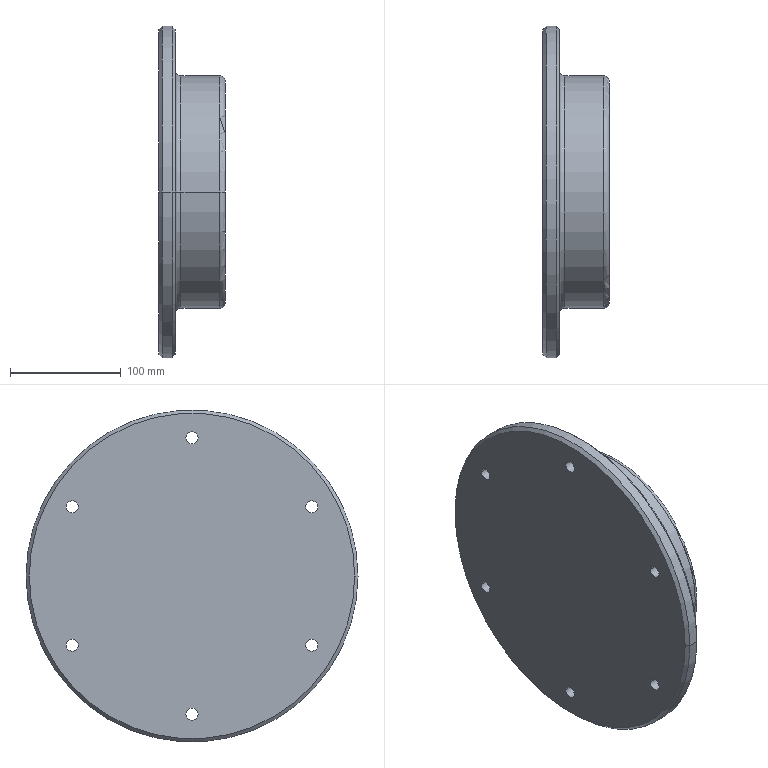Component | SolidWorks | EndCapCover-1 | 1 solid | 39 faces | box 60 x 300 x 300 mm | volume 2597910 mm3 | cone 16 | cylinder 16 | torus 4 | plane 3 | commonest cylinder face diameters 11 x12 210 x2 300 x2
STEP:
#1=COLOUR_RGB('',0.7922,0.8196,0.9333);
#2=FILL_AREA_STYLE_COLOUR('',#1);
#3=FILL_AREA_STYLE('',(#2));
#4=SURFACE_STYLE_FILL_AREA(#3);
#5=SURFACE_SIDE_STYLE('',(#4));
#6=SURFACE_STYLE_USAGE(.BOTH.,#5);
#7=PRESENTATION_STYLE_ASSIGNMENT((#6));
#8=CARTESIAN_POINT('',(4.554,30.148,43.951));
#9=VERTEX_POINT('',#8);
#10=CARTESIAN_POINT('',(4.554,38.416,43.951));
#11=VERTEX_POINT('',#10);
#12=CARTESIAN_POINT('',(4.554,34.282,43.951));
#13=DIRECTION('',(-1.,0.,0.));
#14=DIRECTION('',(0.,1.,0.));
#15=AXIS2_PLACEMENT_3D('',#12,#13,#14);
#16=CIRCLE('',#15,4.134);
#17=EDGE_CURVE('',#9,#11,#16,.T.);
#18=ORIENTED_EDGE('',*,*,#17,.F.);
#19=CARTESIAN_POINT('',(4.751,30.345,43.951));
#20=VERTEX_POINT('',#19);
#21=CARTESIAN_POINT('',(4.554,30.345,43.951));
#22=DIRECTION('',(0.,0.,1.));
#23=DIRECTION('',(0.,-1.,0.));
#24=AXIS2_PLACEMENT_3D('',#21,#22,#23);
#25=CIRCLE('',#24,0.1969);
#26=EDGE_CURVE('',#9,#20,#25,.T.);
#27=ORIENTED_EDGE('',*,*,#26,.T.);
#28=CARTESIAN_POINT('',(4.751,38.219,43.951));
#29=VERTEX_POINT('',#28);
#30=CARTESIAN_POINT('',(4.751,34.282,43.951));
#31=DIRECTION('',(1.,0.,0.));
#32=DIRECTION('',(0.,1.,0.));
#33=AXIS2_PLACEMENT_3D('',#30,#31,#32);
#34=CIRCLE('',#33,3.937);
#35=EDGE_CURVE('',#29,#20,#34,.T.);
#36=ORIENTED_EDGE('',*,*,#35,.F.);
#37=CARTESIAN_POINT('',(4.554,38.219,43.951));
#38=DIRECTION('',(0.,0.,-1.));
#39=DIRECTION('',(-1.,0.,0.));
#40=AXIS2_PLACEMENT_3D('',#37,#38,#39);
#41=CIRCLE('',#40,0.1969);
#42=EDGE_CURVE('',#11,#29,#41,.T.);
#43=ORIENTED_EDGE('',*,*,#42,.F.);
#44=EDGE_LOOP('',(#18,#27,#36,#43));
#45=FACE_OUTER_BOUND('',#44,.T.);
#46=CARTESIAN_POINT('',(4.554,34.282,43.951));
#47=DIRECTION('',(1.,0.,0.));
#48=DIRECTION('',(0.,1.,0.));
#49=AXIS2_PLACEMENT_3D('',#46,#47,#48);
#50=TOROIDAL_SURFACE('',#49,3.937,0.1969);
#51=ADVANCED_FACE('',(#45),#50,.T.);
#52=CARTESIAN_POINT('',(3.176,30.148,43.951));
#53=VERTEX_POINT('',#52);
#54=CARTESIAN_POINT('',(3.176,38.416,43.951));
#55=VERTEX_POINT('',#54);
#56=CARTESIAN_POINT('',(3.176,34.282,43.951));
#57=DIRECTION('',(1.,0.,0.));
#58=DIRECTION('',(0.,1.,0.));
#59=AXIS2_PLACEMENT_3D('',#56,#57,#58);
#60=CIRCLE('',#59,4.134);
#61=EDGE_CURVE('',#53,#55,#60,.T.);
#62=ORIENTED_EDGE('',*,*,#61,.F.);
#63=CARTESIAN_POINT('',(2.979,29.952,43.951));
#64=VERTEX_POINT('',#63);
#65=CARTESIAN_POINT('',(3.176,29.952,43.951));
#66=DIRECTION('',(0.,0.,1.));
#67=DIRECTION('',(0.,-1.,0.));
#68=AXIS2_PLACEMENT_3D('',#65,#66,#67);
#69=CIRCLE('',#68,0.1969);
#70=EDGE_CURVE('',#53,#64,#69,.T.);
#71=ORIENTED_EDGE('',*,*,#70,.T.);
#72=CARTESIAN_POINT('',(2.979,38.613,43.951));
#73=VERTEX_POINT('',#72);
#74=CARTESIAN_POINT('',(2.979,34.282,43.951));
#75=DIRECTION('',(-1.,0.,0.));
#76=DIRECTION('',(0.,1.,0.));
#77=AXIS2_PLACEMENT_3D('',#74,#75,#76);
#78=CIRCLE('',#77,4.331);
#79=EDGE_CURVE('',#73,#64,#78,.T.);
#80=ORIENTED_EDGE('',*,*,#79,.F.);
#81=CARTESIAN_POINT('',(3.176,38.613,43.951));
#82=DIRECTION('',(0.,0.,-1.));
#83=DIRECTION('',(-1.,0.,0.));
#84=AXIS2_PLACEMENT_3D('',#81,#82,#83);
#85=CIRCLE('',#84,0.1969);
#86=EDGE_CURVE('',#55,#73,#85,.T.);
#87=ORIENTED_EDGE('',*,*,#86,.F.);
#88=EDGE_LOOP('',(#62,#71,#80,#87));
#89=FACE_OUTER_BOUND('',#88,.T.);
#90=CARTESIAN_POINT('',(3.176,34.282,43.951));
#91=DIRECTION('',(1.,0.,0.));
#92=DIRECTION('',(0.,1.,0.));
#93=AXIS2_PLACEMENT_3D('',#90,#91,#92);
#94=TOROIDAL_SURFACE('',#93,4.331,0.1969);
#95=ADVANCED_FACE('',(#89),#94,.F.);
#96=CARTESIAN_POINT('',(2.979,40.07,43.951));
#97=VERTEX_POINT('',#96);
#98=CARTESIAN_POINT('',(2.979,28.495,43.951));
#99=VERTEX_POINT('',#98);
#100=CARTESIAN_POINT('',(2.979,34.282,43.951));
#101=DIRECTION('',(1.,0.,0.));
#102=DIRECTION('',(0.,1.,0.));
#103=AXIS2_PLACEMENT_3D('',#100,#101,#102);
#104=CIRCLE('',#103,5.787);
#105=EDGE_CURVE('',#97,#99,#104,.T.);
#106=ORIENTED_EDGE('',*,*,#105,.F.);
#107=CARTESIAN_POINT('',(2.861,40.188,43.951));
#108=VERTEX_POINT('',#107);
#109=CARTESIAN_POINT('',(2.861,40.188,43.951));
#110=DIRECTION('',(-0.7071,0.7071,0.));
#111=VECTOR('',#110,39.37);
#112=LINE('',#109,#111);
#113=EDGE_CURVE('',#97,#108,#112,.T.);
#114=ORIENTED_EDGE('',*,*,#113,.T.);
#115=CARTESIAN_POINT('',(2.861,28.377,43.951));
#116=VERTEX_POINT('',#115);
#117=CARTESIAN_POINT('',(2.861,34.282,43.951));
#118=DIRECTION('',(-1.,0.,0.));
#119=DIRECTION('',(0.,1.,0.));
#120=AXIS2_PLACEMENT_3D('',#117,#118,#119);
#121=CIRCLE('',#120,5.906);
#122=EDGE_CURVE('',#116,#108,#121,.T.);
#123=ORIENTED_EDGE('',*,*,#122,.F.);
#124=CARTESIAN_POINT('',(2.861,28.377,43.951));
#125=DIRECTION('',(-0.7071,-0.7071,0.));
#126=VECTOR('',#125,39.37);
#127=LINE('',#124,#126);
#128=EDGE_CURVE('',#99,#116,#127,.T.);
#129=ORIENTED_EDGE('',*,*,#128,.F.);
#130=EDGE_LOOP('',(#106,#114,#123,#129));
#131=FACE_OUTER_BOUND('',#130,.T.);
#132=CARTESIAN_POINT('',(2.861,34.282,43.951));
#133=DIRECTION('',(-1.,0.,0.));
#134=DIRECTION('',(0.,-1.,0.));
#135=AXIS2_PLACEMENT_3D('',#132,#133,#134);
#136=CONICAL_SURFACE('',#135,5.906,0.7854);
#137=ADVANCED_FACE('',(#131),#136,.T.);
#138=CARTESIAN_POINT('',(2.388,28.495,43.951));
#139=VERTEX_POINT('',#138);
#140=CARTESIAN_POINT('',(2.388,40.07,43.951));
#141=VERTEX_POINT('',#140);
#142=CARTESIAN_POINT('',(2.388,34.282,43.951));
#143=DIRECTION('',(-1.,0.,0.));
#144=DIRECTION('',(0.,-1.,0.));
#145=AXIS2_PLACEMENT_3D('',#142,#143,#144);
#146=CIRCLE('',#145,5.787);
#147=EDGE_CURVE('',#139,#141,#146,.T.);
#148=ORIENTED_EDGE('',*,*,#147,.F.);
#149=CARTESIAN_POINT('',(2.507,28.377,43.951));
#150=VERTEX_POINT('',#149);
#151=CARTESIAN_POINT('',(2.388,28.495,43.951));
#152=DIRECTION('',(0.7071,-0.7071,0.));
#153=VECTOR('',#152,39.37);
#154=LINE('',#151,#153);
#155=EDGE_CURVE('',#139,#150,#154,.T.);
#156=ORIENTED_EDGE('',*,*,#155,.T.);
#157=CARTESIAN_POINT('',(2.507,40.188,43.951));
#158=VERTEX_POINT('',#157);
#159=CARTESIAN_POINT('',(2.507,34.282,43.951));
#160=DIRECTION('',(1.,0.,0.));
#161=DIRECTION('',(0.,-1.,0.));
#162=AXIS2_PLACEMENT_3D('',#159,#160,#161);
#163=CIRCLE('',#162,5.906);
#164=EDGE_CURVE('',#158,#150,#163,.T.);
#165=ORIENTED_EDGE('',*,*,#164,.F.);
#166=CARTESIAN_POINT('',(2.388,40.07,43.951));
#167=DIRECTION('',(0.7071,0.7071,0.));
#168=VECTOR('',#167,39.37);
#169=LINE('',#166,#168);
#170=EDGE_CURVE('',#141,#158,#169,.T.);
#171=ORIENTED_EDGE('',*,*,#170,.F.);
#172=EDGE_LOOP('',(#148,#156,#165,#171));
#173=FACE_OUTER_BOUND('',#172,.T.);
#174=CARTESIAN_POINT('',(2.388,34.282,43.951));
#175=DIRECTION('',(1.,0.,0.));
#176=DIRECTION('',(0.,1.,0.));
#177=AXIS2_PLACEMENT_3D('',#174,#175,#176);
#178=CONICAL_SURFACE('',#177,5.787,0.7854);
#179=ADVANCED_FACE('',(#173),#178,.T.);
#180=CARTESIAN_POINT('',(2.764,38.322,46.408));
#181=VERTEX_POINT('',#180);
#182=CARTESIAN_POINT('',(2.764,38.755,46.408));
#183=VERTEX_POINT('',#182);
#184=CARTESIAN_POINT('',(2.764,38.538,46.408));
#185=DIRECTION('',(1.,0.,0.));
#186=DIRECTION('',(0.,1.,0.));
#187=AXIS2_PLACEMENT_3D('',#184,#185,#186);
#188=CIRCLE('',#187,0.2165);
#189=EDGE_CURVE('',#181,#183,#188,.T.);
#190=ORIENTED_EDGE('',*,*,#189,.F.);
#191=CARTESIAN_POINT('',(2.979,38.107,46.408));
#192=VERTEX_POINT('',#191);
#193=CARTESIAN_POINT('',(2.764,38.322,46.408));
#194=DIRECTION('',(0.7071,-0.7071,0.));
#195=VECTOR('',#194,39.37);
#196=LINE('',#193,#195);
#197=EDGE_CURVE('',#181,#192,#196,.T.);
#198=ORIENTED_EDGE('',*,*,#197,.T.);
#199=CARTESIAN_POINT('',(2.979,38.969,46.408));
#200=VERTEX_POINT('',#199);
#201=CARTESIAN_POINT('',(2.979,38.538,46.408));
#202=DIRECTION('',(-1.,0.,0.));
#203=DIRECTION('',(0.,1.,0.));
#204=AXIS2_PLACEMENT_3D('',#201,#202,#203);
#205=CIRCLE('',#204,0.4311);
#206=EDGE_CURVE('',#200,#192,#205,.T.);
#207=ORIENTED_EDGE('',*,*,#206,.F.);
#208=CARTESIAN_POINT('',(2.764,38.755,46.408));
#209=DIRECTION('',(0.7071,0.7071,0.));
#210=VECTOR('',#209,39.37);
#211=LINE('',#208,#210);
#212=EDGE_CURVE('',#183,#200,#211,.T.);
#213=ORIENTED_EDGE('',*,*,#212,.F.);
#214=EDGE_LOOP('',(#190,#198,#207,#213));
#215=FACE_OUTER_BOUND('',#214,.T.);
#216=CARTESIAN_POINT('',(2.764,38.538,46.408));
#217=DIRECTION('',(1.,0.,0.));
#218=DIRECTION('',(0.,1.,0.));
#219=AXIS2_PLACEMENT_3D('',#216,#217,#218);
#220=CONICAL_SURFACE('',#219,0.2165,0.7854);
#221=ADVANCED_FACE('',(#215),#220,.F.);
#222=CARTESIAN_POINT('',(2.764,34.066,48.865));
#223=VERTEX_POINT('',#222);
#224=CARTESIAN_POINT('',(2.764,34.499,48.865));
#225=VERTEX_POINT('',#224);
#226=CARTESIAN_POINT('',(2.764,34.282,48.865));
#227=DIRECTION('',(1.,0.,0.));
#228=DIRECTION('',(0.,1.,0.));
#229=AXIS2_PLACEMENT_3D('',#226,#227,#228);
#230=CIRCLE('',#229,0.2165);
#231=EDGE_CURVE('',#223,#225,#230,.T.);
#232=ORIENTED_EDGE('',*,*,#231,.F.);
#233=CARTESIAN_POINT('',(2.979,33.851,48.865));
#234=VERTEX_POINT('',#233);
#235=CARTESIAN_POINT('',(2.764,34.066,48.865));
#236=DIRECTION('',(0.7071,-0.7071,0.));
#237=VECTOR('',#236,39.37);
#238=LINE('',#235,#237);
#239=EDGE_CURVE('',#223,#234,#238,.T.);
#240=ORIENTED_EDGE('',*,*,#239,.T.);
#241=CARTESIAN_POINT('',(2.979,34.713,48.865));
#242=VERTEX_POINT('',#241);
#243=CARTESIAN_POINT('',(2.979,34.282,48.865));
#244=DIRECTION('',(-1.,0.,0.));
#245=DIRECTION('',(0.,1.,0.));
#246=AXIS2_PLACEMENT_3D('',#243,#244,#245);
#247=CIRCLE('',#246,0.4311);
#248=EDGE_CURVE('',#242,#234,#247,.T.);
#249=ORIENTED_EDGE('',*,*,#248,.F.);
#250=CARTESIAN_POINT('',(2.764,34.499,48.865));
#251=DIRECTION('',(0.7071,0.7071,0.));
#252=VECTOR('',#251,39.37);
#253=LINE('',#250,#252);
#254=EDGE_CURVE('',#225,#242,#253,.T.);
#255=ORIENTED_EDGE('',*,*,#254,.F.);
#256=EDGE_LOOP('',(#232,#240,#249,#255));
#257=FACE_OUTER_BOUND('',#256,.T.);
#258=CARTESIAN_POINT('',(2.764,34.282,48.865));
#259=DIRECTION('',(1.,0.,0.));
#260=DIRECTION('',(0.,1.,0.));
#261=AXIS2_PLACEMENT_3D('',#258,#259,#260);
#262=CONICAL_SURFACE('',#261,0.2165,0.7854);
#263=ADVANCED_FACE('',(#257),#262,.F.);
#264=CARTESIAN_POINT('',(2.764,29.81,41.494));
#265=VERTEX_POINT('',#264);
#266=CARTESIAN_POINT('',(2.764,30.243,41.494));
#267=VERTEX_POINT('',#266);
#268=CARTESIAN_POINT('',(2.764,30.026,41.494));
#269=DIRECTION('',(1.,0.,0.));
#270=DIRECTION('',(0.,1.,0.));
#271=AXIS2_PLACEMENT_3D('',#268,#269,#270);
#272=CIRCLE('',#271,0.2165);
#273=EDGE_CURVE('',#265,#267,#272,.T.);
#274=ORIENTED_EDGE('',*,*,#273,.F.);
#275=CARTESIAN_POINT('',(2.979,29.595,41.494));
#276=VERTEX_POINT('',#275);
#277=CARTESIAN_POINT('',(2.764,29.81,41.494));
#278=DIRECTION('',(0.7071,-0.7071,0.));
#279=VECTOR('',#278,39.37);
#280=LINE('',#277,#279);
#281=EDGE_CURVE('',#265,#276,#280,.T.);
#282=ORIENTED_EDGE('',*,*,#281,.T.);
#283=CARTESIAN_POINT('',(2.979,30.457,41.494));
#284=VERTEX_POINT('',#283);
#285=CARTESIAN_POINT('',(2.979,30.026,41.494));
#286=DIRECTION('',(-1.,0.,0.));
#287=DIRECTION('',(0.,1.,0.));
#288=AXIS2_PLACEMENT_3D('',#285,#286,#287);
#289=CIRCLE('',#288,0.4311);
#290=EDGE_CURVE('',#284,#276,#289,.T.);
#291=ORIENTED_EDGE('',*,*,#290,.F.);
#292=CARTESIAN_POINT('',(2.764,30.243,41.494));
#293=DIRECTION('',(0.7071,0.7071,0.));
#294=VECTOR('',#293,39.37);
#295=LINE('',#292,#294);
#296=EDGE_CURVE('',#267,#284,#295,.T.);
#297=ORIENTED_EDGE('',*,*,#296,.F.);
#298=EDGE_LOOP('',(#274,#282,#291,#297));
#299=FACE_OUTER_BOUND('',#298,.T.);
#300=CARTESIAN_POINT('',(2.764,30.026,41.494));
#301=DIRECTION('',(1.,0.,0.));
#302=DIRECTION('',(0.,1.,0.));
#303=AXIS2_PLACEMENT_3D('',#300,#301,#302);
#304=CONICAL_SURFACE('',#303,0.2165,0.7854);
#305=ADVANCED_FACE('',(#299),#304,.F.);
#306=CARTESIAN_POINT('',(2.764,34.066,39.036));
#307=VERTEX_POINT('',#306);
#308=CARTESIAN_POINT('',(2.764,34.499,39.036));
#309=VERTEX_POINT('',#308);
#310=CARTESIAN_POINT('',(2.764,34.282,39.036));
#311=DIRECTION('',(1.,0.,0.));
#312=DIRECTION('',(0.,1.,0.));
#313=AXIS2_PLACEMENT_3D('',#310,#311,#312);
#314=CIRCLE('',#313,0.2165);
#315=EDGE_CURVE('',#307,#309,#314,.T.);
#316=ORIENTED_EDGE('',*,*,#315,.F.);
#317=CARTESIAN_POINT('',(2.979,33.851,39.036));
#318=VERTEX_POINT('',#317);
#319=CARTESIAN_POINT('',(2.764,34.066,39.036));
#320=DIRECTION('',(0.7071,-0.7071,0.));
#321=VECTOR('',#320,39.37);
#322=LINE('',#319,#321);
#323=EDGE_CURVE('',#307,#318,#322,.T.);
#324=ORIENTED_EDGE('',*,*,#323,.T.);
#325=CARTESIAN_POINT('',(2.979,34.713,39.036));
#326=VERTEX_POINT('',#325);
#327=CARTESIAN_POINT('',(2.979,34.282,39.036));
#328=DIRECTION('',(-1.,0.,0.));
#329=DIRECTION('',(0.,1.,0.));
#330=AXIS2_PLACEMENT_3D('',#327,#328,#329);
#331=CIRCLE('',#330,0.4311);
#332=EDGE_CURVE('',#326,#318,#331,.T.);
#333=ORIENTED_EDGE('',*,*,#332,.F.);
#334=CARTESIAN_POINT('',(2.764,34.499,39.036));
#335=DIRECTION('',(0.7071,0.7071,0.));
#336=VECTOR('',#335,39.37);
#337=LINE('',#334,#336);
#338=EDGE_CURVE('',#309,#326,#337,.T.);
#339=ORIENTED_EDGE('',*,*,#338,.F.);
#340=EDGE_LOOP('',(#316,#324,#333,#339));
#341=FACE_OUTER_BOUND('',#340,.T.);
#342=CARTESIAN_POINT('',(2.764,34.282,39.036));
#343=DIRECTION('',(1.,0.,0.));
#344=DIRECTION('',(0.,1.,0.));
#345=AXIS2_PLACEMENT_3D('',#342,#343,#344);
#346=CONICAL_SURFACE('',#345,0.2165,0.7854);
#347=ADVANCED_FACE('',(#341),#346,.F.);
#348=CARTESIAN_POINT('',(2.764,29.81,46.408));
#349=VERTEX_POINT('',#348);
#350=CARTESIAN_POINT('',(2.764,30.243,46.408));
#351=VERTEX_POINT('',#350);
#352=CARTESIAN_POINT('',(2.764,30.026,46.408));
#353=DIRECTION('',(1.,0.,0.));
#354=DIRECTION('',(0.,1.,0.));
#355=AXIS2_PLACEMENT_3D('',#352,#353,#354);
#356=CIRCLE('',#355,0.2165);
#357=EDGE_CURVE('',#349,#351,#356,.T.);
#358=ORIENTED_EDGE('',*,*,#357,.F.);
#359=CARTESIAN_POINT('',(2.979,29.595,46.408));
#360=VERTEX_POINT('',#359);
#361=CARTESIAN_POINT('',(2.764,29.81,46.408));
#362=DIRECTION('',(0.7071,-0.7071,0.));
#363=VECTOR('',#362,39.37);
#364=LINE('',#361,#363);
#365=EDGE_CURVE('',#349,#360,#364,.T.);
#366=ORIENTED_EDGE('',*,*,#365,.T.);
#367=CARTESIAN_POINT('',(2.979,30.457,46.408));
#368=VERTEX_POINT('',#367);
#369=CARTESIAN_POINT('',(2.979,30.026,46.408));
#370=DIRECTION('',(-1.,0.,0.));
#371=DIRECTION('',(0.,1.,0.));
#372=AXIS2_PLACEMENT_3D('',#369,#370,#371);
#373=CIRCLE('',#372,0.4311);
#374=EDGE_CURVE('',#368,#360,#373,.T.);
#375=ORIENTED_EDGE('',*,*,#374,.F.);
#376=CARTESIAN_POINT('',(2.764,30.243,46.408));
#377=DIRECTION('',(0.7071,0.7071,0.));
#378=VECTOR('',#377,39.37);
#379=LINE('',#376,#378);
#380=EDGE_CURVE('',#351,#368,#379,.T.);
#381=ORIENTED_EDGE('',*,*,#380,.F.);
#382=EDGE_LOOP('',(#358,#366,#375,#381));
#383=FACE_OUTER_BOUND('',#382,.T.);
#384=CARTESIAN_POINT('',(2.764,30.026,46.408));
#385=DIRECTION('',(1.,0.,0.));
#386=DIRECTION('',(0.,1.,0.));
#387=AXIS2_PLACEMENT_3D('',#384,#385,#386);
#388=CONICAL_SURFACE('',#387,0.2165,0.7854);
#389=ADVANCED_FACE('',(#383),#388,.F.);
#390=CARTESIAN_POINT('',(2.764,38.322,41.494));
#391=VERTEX_POINT('',#390);
#392=CARTESIAN_POINT('',(2.764,38.755,41.494));
#393=VERTEX_POINT('',#392);
#394=CARTESIAN_POINT('',(2.764,38.538,41.494));
#395=DIRECTION('',(1.,0.,0.));
#396=DIRECTION('',(0.,1.,0.));
#397=AXIS2_PLACEMENT_3D('',#394,#395,#396);
#398=CIRCLE('',#397,0.2165);
#399=EDGE_CURVE('',#391,#393,#398,.T.);
#400=ORIENTED_EDGE('',*,*,#399,.F.);
#401=CARTESIAN_POINT('',(2.979,38.107,41.494));
#402=VERTEX_POINT('',#401);
#403=CARTESIAN_POINT('',(2.764,38.322,41.494));
#404=DIRECTION('',(0.7071,-0.7071,0.));
#405=VECTOR('',#404,39.37);
#406=LINE('',#403,#405);
#407=EDGE_CURVE('',#391,#402,#406,.T.);
#408=ORIENTED_EDGE('',*,*,#407,.T.);
#409=CARTESIAN_POINT('',(2.979,38.969,41.494));
#410=VERTEX_POINT('',#409);
#411=CARTESIAN_POINT('',(2.979,38.538,41.494));
#412=DIRECTION('',(-1.,0.,0.));
#413=DIRECTION('',(0.,1.,0.));
#414=AXIS2_PLACEMENT_3D('',#411,#412,#413);
#415=CIRCLE('',#414,0.4311);
#416=EDGE_CURVE('',#410,#402,#415,.T.);
#417=ORIENTED_EDGE('',*,*,#416,.F.);
#418=CARTESIAN_POINT('',(2.764,38.755,41.494));
#419=DIRECTION('',(0.7071,0.7071,0.));
#420=VECTOR('',#419,39.37);
#421=LINE('',#418,#420);
#422=EDGE_CURVE('',#393,#410,#421,.T.);
#423=ORIENTED_EDGE('',*,*,#422,.F.);
#424=EDGE_LOOP('',(#400,#408,#417,#423));
#425=FACE_OUTER_BOUND('',#424,.T.);
#426=CARTESIAN_POINT('',(2.764,38.538,41.494));
#427=DIRECTION('',(1.,0.,0.));
#428=DIRECTION('',(0.,1.,0.));
#429=AXIS2_PLACEMENT_3D('',#426,#427,#428);
#430=CONICAL_SURFACE('',#429,0.2165,0.7854);
#431=ADVANCED_FACE('',(#425),#430,.F.);
#432=CARTESIAN_POINT('',(2.388,29.81,41.494));
#433=VERTEX_POINT('',#432);
#434=CARTESIAN_POINT('',(2.388,30.243,41.494));
#435=VERTEX_POINT('',#434);
#436=CARTESIAN_POINT('',(2.388,30.026,41.494));
#437=DIRECTION('',(1.,0.,0.));
#438=DIRECTION('',(0.,1.,0.));
#439=AXIS2_PLACEMENT_3D('',#436,#437,#438);
#440=CIRCLE('',#439,0.2165);
#441=EDGE_CURVE('',#433,#435,#440,.T.);
#442=ORIENTED_EDGE('',*,*,#441,.F.);
#443=CARTESIAN_POINT('',(2.979,29.81,41.494));
#444=DIRECTION('',(1.,0.,0.));
#445=VECTOR('',#444,39.37);
#446=LINE('',#443,#445);
#447=EDGE_CURVE('',#433,#265,#446,.T.);
#448=ORIENTED_EDGE('',*,*,#447,.T.);
#449=ORIENTED_EDGE('',*,*,#273,.T.);
#450=CARTESIAN_POINT('',(2.979,30.243,41.494));
#451=DIRECTION('',(1.,0.,0.));
#452=VECTOR('',#451,39.37);
#453=LINE('',#450,#452);
#454=EDGE_CURVE('',#435,#267,#453,.T.);
#455=ORIENTED_EDGE('',*,*,#454,.F.);
#456=EDGE_LOOP('',(#442,#448,#449,#455));
#457=FACE_OUTER_BOUND('',#456,.T.);
#458=CARTESIAN_POINT('',(2.979,30.026,41.494));
#459=DIRECTION('',(1.,0.,0.));
#460=DIRECTION('',(0.,1.,0.));
#461=AXIS2_PLACEMENT_3D('',#458,#459,#460);
#462=CYLINDRICAL_SURFACE('',#461,0.2165);
#463=ADVANCED_FACE('',(#457),#462,.F.);
#464=CARTESIAN_POINT('',(2.388,29.81,46.408));
#465=VERTEX_POINT('',#464);
#466=CARTESIAN_POINT('',(2.388,30.243,46.408));
#467=VERTEX_POINT('',#466);
#468=CARTESIAN_POINT('',(2.388,30.026,46.408));
#469=DIRECTION('',(1.,0.,0.));
#470=DIRECTION('',(0.,1.,0.));
#471=AXIS2_PLACEMENT_3D('',#468,#469,#470);
#472=CIRCLE('',#471,0.2165);
#473=EDGE_CURVE('',#465,#467,#472,.T.);
#474=ORIENTED_EDGE('',*,*,#473,.F.);
#475=CARTESIAN_POINT('',(2.979,29.81,46.408));
#476=DIRECTION('',(1.,0.,0.));
#477=VECTOR('',#476,39.37);
#478=LINE('',#475,#477);
#479=EDGE_CURVE('',#465,#349,#478,.T.);
#480=ORIENTED_EDGE('',*,*,#479,.T.);
#481=ORIENTED_EDGE('',*,*,#357,.T.);
#482=CARTESIAN_POINT('',(2.979,30.243,46.408));
#483=DIRECTION('',(1.,0.,0.));
#484=VECTOR('',#483,39.37);
#485=LINE('',#482,#484);
#486=EDGE_CURVE('',#467,#351,#485,.T.);
#487=ORIENTED_EDGE('',*,*,#486,.F.);
#488=EDGE_LOOP('',(#474,#480,#481,#487));
#489=FACE_OUTER_BOUND('',#488,.T.);
#490=CARTESIAN_POINT('',(2.979,30.026,46.408));
#491=DIRECTION('',(1.,0.,0.));
#492=DIRECTION('',(0.,1.,0.));
#493=AXIS2_PLACEMENT_3D('',#490,#491,#492);
#494=CYLINDRICAL_SURFACE('',#493,0.2165);
#495=ADVANCED_FACE('',(#489),#494,.F.);
#496=CARTESIAN_POINT('',(2.388,34.066,48.865));
#497=VERTEX_POINT('',#496);
#498=CARTESIAN_POINT('',(2.388,34.499,48.865));
#499=VERTEX_POINT('',#498);
#500=CARTESIAN_POINT('',(2.388,34.282,48.865));
#501=DIRECTION('',(1.,0.,0.));
#502=DIRECTION('',(0.,1.,0.));
#503=AXIS2_PLACEMENT_3D('',#500,#501,#502);
#504=CIRCLE('',#503,0.2165);
#505=EDGE_CURVE('',#497,#499,#504,.T.);
#506=ORIENTED_EDGE('',*,*,#505,.F.);
#507=CARTESIAN_POINT('',(2.979,34.066,48.865));
#508=DIRECTION('',(1.,0.,0.));
#509=VECTOR('',#508,39.37);
#510=LINE('',#507,#509);
#511=EDGE_CURVE('',#497,#223,#510,.T.);
#512=ORIENTED_EDGE('',*,*,#511,.T.);
#513=ORIENTED_EDGE('',*,*,#231,.T.);
#514=CARTESIAN_POINT('',(2.979,34.499,48.865));
#515=DIRECTION('',(1.,0.,0.));
#516=VECTOR('',#515,39.37);
#517=LINE('',#514,#516);
#518=EDGE_CURVE('',#499,#225,#517,.T.);
#519=ORIENTED_EDGE('',*,*,#518,.F.);
#520=EDGE_LOOP('',(#506,#512,#513,#519));
#521=FACE_OUTER_BOUND('',#520,.T.);
#522=CARTESIAN_POINT('',(2.979,34.282,48.865));
#523=DIRECTION('',(1.,0.,0.));
#524=DIRECTION('',(0.,1.,0.));
#525=AXIS2_PLACEMENT_3D('',#522,#523,#524);
#526=CYLINDRICAL_SURFACE('',#525,0.2165);
#527=ADVANCED_FACE('',(#521),#526,.F.);
#528=CARTESIAN_POINT('',(2.388,38.322,46.408));
#529=VERTEX_POINT('',#528);
#530=CARTESIAN_POINT('',(2.388,38.755,46.408));
#531=VERTEX_POINT('',#530);
#532=CARTESIAN_POINT('',(2.388,38.538,46.408));
#533=DIRECTION('',(1.,0.,0.));
#534=DIRECTION('',(0.,1.,0.));
#535=AXIS2_PLACEMENT_3D('',#532,#533,#534);
#536=CIRCLE('',#535,0.2165);
#537=EDGE_CURVE('',#529,#531,#536,.T.);
#538=ORIENTED_EDGE('',*,*,#537,.F.);
#539=CARTESIAN_POINT('',(2.979,38.322,46.408));
#540=DIRECTION('',(1.,0.,0.));
#541=VECTOR('',#540,39.37);
#542=LINE('',#539,#541);
#543=EDGE_CURVE('',#529,#181,#542,.T.);
#544=ORIENTED_EDGE('',*,*,#543,.T.);
#545=ORIENTED_EDGE('',*,*,#189,.T.);
#546=CARTESIAN_POINT('',(2.979,38.755,46.408));
#547=DIRECTION('',(1.,0.,0.));
#548=VECTOR('',#547,39.37);
#549=LINE('',#546,#548);
#550=EDGE_CURVE('',#531,#183,#549,.T.);
#551=ORIENTED_EDGE('',*,*,#550,.F.);
#552=EDGE_LOOP('',(#538,#544,#545,#551));
#553=FACE_OUTER_BOUND('',#552,.T.);
#554=CARTESIAN_POINT('',(2.979,38.538,46.408));
#555=DIRECTION('',(1.,0.,0.));
#556=DIRECTION('',(0.,1.,0.));
#557=AXIS2_PLACEMENT_3D('',#554,#555,#556);
#558=CYLINDRICAL_SURFACE('',#557,0.2165);
#559=ADVANCED_FACE('',(#553),#558,.F.);
#560=CARTESIAN_POINT('',(2.388,38.322,41.494));
#561=VERTEX_POINT('',#560);
#562=CARTESIAN_POINT('',(2.388,38.755,41.494));
#563=VERTEX_POINT('',#562);
#564=CARTESIAN_POINT('',(2.388,38.538,41.494));
#565=DIRECTION('',(1.,0.,0.));
#566=DIRECTION('',(0.,1.,0.));
#567=AXIS2_PLACEMENT_3D('',#564,#565,#566);
#568=CIRCLE('',#567,0.2165);
#569=EDGE_CURVE('',#561,#563,#568,.T.);
#570=ORIENTED_EDGE('',*,*,#569,.F.);
#571=CARTESIAN_POINT('',(2.979,38.322,41.494));
#572=DIRECTION('',(1.,0.,0.));
#573=VECTOR('',#572,39.37);
#574=LINE('',#571,#573);
#575=EDGE_CURVE('',#561,#391,#574,.T.);
#576=ORIENTED_EDGE('',*,*,#575,.T.);
#577=ORIENTED_EDGE('',*,*,#399,.T.);
#578=CARTESIAN_POINT('',(2.979,38.755,41.494));
#579=DIRECTION('',(1.,0.,0.));
#580=VECTOR('',#579,39.37);
#581=LINE('',#578,#580);
#582=EDGE_CURVE('',#563,#393,#581,.T.);
#583=ORIENTED_EDGE('',*,*,#582,.F.);
#584=EDGE_LOOP('',(#570,#576,#577,#583));
#585=FACE_OUTER_BOUND('',#584,.T.);
#586=CARTESIAN_POINT('',(2.979,38.538,41.494));
#587=DIRECTION('',(1.,0.,0.));
#588=DIRECTION('',(0.,1.,0.));
#589=AXIS2_PLACEMENT_3D('',#586,#587,#588);
#590=CYLINDRICAL_SURFACE('',#589,0.2165);
#591=ADVANCED_FACE('',(#585),#590,.F.);
#592=CARTESIAN_POINT('',(2.388,34.066,39.036));
#593=VERTEX_POINT('',#592);
#594=CARTESIAN_POINT('',(2.388,34.499,39.036));
#595=VERTEX_POINT('',#594);
#596=CARTESIAN_POINT('',(2.388,34.282,39.036));
#597=DIRECTION('',(1.,0.,0.));
#598=DIRECTION('',(0.,1.,0.));
#599=AXIS2_PLACEMENT_3D('',#596,#597,#598);
#600=CIRCLE('',#599,0.2165);
#601=EDGE_CURVE('',#593,#595,#600,.T.);
#602=ORIENTED_EDGE('',*,*,#601,.F.);
#603=CARTESIAN_POINT('',(2.979,34.066,39.036));
#604=DIRECTION('',(1.,0.,0.));
#605=VECTOR('',#604,39.37);
#606=LINE('',#603,#605);
#607=EDGE_CURVE('',#593,#307,#606,.T.);
#608=ORIENTED_EDGE('',*,*,#607,.T.);
#609=ORIENTED_EDGE('',*,*,#315,.T.);
#610=CARTESIAN_POINT('',(2.979,34.499,39.036));
#611=DIRECTION('',(1.,0.,0.));
#612=VECTOR('',#611,39.37);
#613=LINE('',#610,#612);
#614=EDGE_CURVE('',#595,#309,#613,.T.);
#615=ORIENTED_EDGE('',*,*,#614,.F.);
#616=EDGE_LOOP('',(#602,#608,#609,#615));
#617=FACE_OUTER_BOUND('',#616,.T.);
#618=CARTESIAN_POINT('',(2.979,34.282,39.036));
#619=DIRECTION('',(1.,0.,0.));
#620=DIRECTION('',(0.,1.,0.));
#621=AXIS2_PLACEMENT_3D('',#618,#619,#620);
#622=CYLINDRICAL_SURFACE('',#621,0.2165);
#623=ADVANCED_FACE('',(#617),#622,.F.);
#624=ORIENTED_EDGE('',*,*,#17,.T.);
#625=CARTESIAN_POINT('',(4.751,38.416,43.951));
#626=DIRECTION('',(-1.,0.,0.));
#627=VECTOR('',#626,39.37);
#628=LINE('',#625,#627);
#629=EDGE_CURVE('',#11,#55,#628,.T.);
#630=ORIENTED_EDGE('',*,*,#629,.T.);
#631=CARTESIAN_POINT('',(3.176,34.282,43.951));
#632=DIRECTION('',(1.,0.,0.));
#633=DIRECTION('',(0.,1.,0.));
#634=AXIS2_PLACEMENT_3D('',#631,#632,#633);
#635=CIRCLE('',#634,4.134);
#636=EDGE_CURVE('',#55,#53,#635,.T.);
#637=ORIENTED_EDGE('',*,*,#636,.T.);
#638=CARTESIAN_POINT('',(4.751,30.148,43.951));
#639=DIRECTION('',(-1.,0.,0.));
#640=VECTOR('',#639,39.37);
#641=LINE('',#638,#640);
#642=EDGE_CURVE('',#9,#53,#641,.T.);
#643=ORIENTED_EDGE('',*,*,#642,.F.);
#644=EDGE_LOOP('',(#624,#630,#637,#643));
#645=FACE_OUTER_BOUND('',#644,.T.);
#646=CARTESIAN_POINT('',(4.751,34.282,43.951));
#647=DIRECTION('',(-1.,0.,0.));
#648=DIRECTION('',(0.,-1.,0.));
#649=AXIS2_PLACEMENT_3D('',#646,#647,#648);
#650=CYLINDRICAL_SURFACE('',#649,4.134);
#651=ADVANCED_FACE('',(#645),#650,.T.);
#652=ORIENTED_EDGE('',*,*,#122,.T.);
#653=CARTESIAN_POINT('',(2.979,40.188,43.951));
#654=DIRECTION('',(-1.,0.,0.));
#655=VECTOR('',#654,39.37);
#656=LINE('',#653,#655);
#657=EDGE_CURVE('',#108,#158,#656,.T.);
#658=ORIENTED_EDGE('',*,*,#657,.T.);
#659=ORIENTED_EDGE('',*,*,#164,.T.);
#660=CARTESIAN_POINT('',(2.979,28.377,43.951));
#661=DIRECTION('',(-1.,0.,0.));
#662=VECTOR('',#661,39.37);
#663=LINE('',#660,#662);
#664=EDGE_CURVE('',#116,#150,#663,.T.);
#665=ORIENTED_EDGE('',*,*,#664,.F.);
#666=EDGE_LOOP('',(#652,#658,#659,#665));
#667=FACE_OUTER_BOUND('',#666,.T.);
#668=CARTESIAN_POINT('',(2.979,34.282,43.951));
#669=DIRECTION('',(-1.,0.,0.));
#670=DIRECTION('',(0.,-1.,0.));
#671=AXIS2_PLACEMENT_3D('',#668,#669,#670);
#672=CYLINDRICAL_SURFACE('',#671,5.906);
#673=ADVANCED_FACE('',(#667),#672,.T.);
#674=ORIENTED_EDGE('',*,*,#657,.F.);
#675=CARTESIAN_POINT('',(2.861,34.282,43.951));
#676=DIRECTION('',(-1.,0.,0.));
#677=DIRECTION('',(0.,1.,0.));
#678=AXIS2_PLACEMENT_3D('',#675,#676,#677);
#679=CIRCLE('',#678,5.906);
#680=EDGE_CURVE('',#108,#116,#679,.T.);
#681=ORIENTED_EDGE('',*,*,#680,.T.);
#682=ORIENTED_EDGE('',*,*,#664,.T.);
#683=CARTESIAN_POINT('',(2.507,34.282,43.951));
#684=DIRECTION('',(1.,0.,0.));
#685=DIRECTION('',(0.,-1.,0.));
#686=AXIS2_PLACEMENT_3D('',#683,#684,#685);
#687=CIRCLE('',#686,5.906);
#688=EDGE_CURVE('',#150,#158,#687,.T.);
#689=ORIENTED_EDGE('',*,*,#688,.T.);
#690=EDGE_LOOP('',(#674,#681,#682,#689));
#691=FACE_OUTER_BOUND('',#690,.T.);
#692=CARTESIAN_POINT('',(2.979,34.282,43.951));
#693=DIRECTION('',(-1.,0.,0.));
#694=DIRECTION('',(0.,-1.,0.));
#695=AXIS2_PLACEMENT_3D('',#692,#693,#694);
#696=CYLINDRICAL_SURFACE('',#695,5.906);
#697=ADVANCED_FACE('',(#691),#696,.T.);
#698=ORIENTED_EDGE('',*,*,#79,.T.);
#699=CARTESIAN_POINT('',(2.979,34.282,43.951));
#700=DIRECTION('',(-1.,0.,0.));
#701=DIRECTION('',(0.,1.,0.));
#702=AXIS2_PLACEMENT_3D('',#699,#700,#701);
#703=CIRCLE('',#702,4.331);
#704=EDGE_CURVE('',#64,#73,#703,.T.);
#705=ORIENTED_EDGE('',*,*,#704,.T.);
#706=EDGE_LOOP('',(#698,#705));
#707=FACE_BOUND('',#706,.T.);
#708=CARTESIAN_POINT('',(2.979,34.282,43.951));
#709=DIRECTION('',(1.,0.,0.));
#710=DIRECTION('',(0.,1.,0.));
#711=AXIS2_PLACEMENT_3D('',#708,#709,#710);
#712=CIRCLE('',#711,5.787);
#713=EDGE_CURVE('',#99,#97,#712,.T.);
#714=ORIENTED_EDGE('',*,*,#713,.T.);
#715=ORIENTED_EDGE('',*,*,#105,.T.);
#716=EDGE_LOOP('',(#714,#715));
#717=FACE_OUTER_BOUND('',#716,.T.);
#718=ORIENTED_EDGE('',*,*,#416,.T.);
#719=CARTESIAN_POINT('',(2.979,38.538,41.494));
#720=DIRECTION('',(-1.,0.,0.));
#721=DIRECTION('',(0.,1.,0.));
#722=AXIS2_PLACEMENT_3D('',#719,#720,#721);
#723=CIRCLE('',#722,0.4311);
#724=EDGE_CURVE('',#402,#410,#723,.T.);
#725=ORIENTED_EDGE('',*,*,#724,.T.);
#726=EDGE_LOOP('',(#718,#725));
#727=FACE_BOUND('',#726,.T.);
#728=ORIENTED_EDGE('',*,*,#374,.T.);
#729=CARTESIAN_POINT('',(2.979,30.026,46.408));
#730=DIRECTION('',(-1.,0.,0.));
#731=DIRECTION('',(0.,1.,0.));
#732=AXIS2_PLACEMENT_3D('',#729,#730,#731);
#733=CIRCLE('',#732,0.4311);
#734=EDGE_CURVE('',#360,#368,#733,.T.);
#735=ORIENTED_EDGE('',*,*,#734,.T.);
#736=EDGE_LOOP('',(#728,#735));
#737=FACE_BOUND('',#736,.T.);
#738=ORIENTED_EDGE('',*,*,#332,.T.);
#739=CARTESIAN_POINT('',(2.979,34.282,39.036));
#740=DIRECTION('',(-1.,0.,0.));
#741=DIRECTION('',(0.,1.,0.));
#742=AXIS2_PLACEMENT_3D('',#739,#740,#741);
#743=CIRCLE('',#742,0.4311);
#744=EDGE_CURVE('',#318,#326,#743,.T.);
#745=ORIENTED_EDGE('',*,*,#744,.T.);
#746=EDGE_LOOP('',(#738,#745));
#747=FACE_BOUND('',#746,.T.);
#748=ORIENTED_EDGE('',*,*,#290,.T.);
#749=CARTESIAN_POINT('',(2.979,30.026,41.494));
#750=DIRECTION('',(-1.,0.,0.));
#751=DIRECTION('',(0.,1.,0.));
#752=AXIS2_PLACEMENT_3D('',#749,#750,#751);
#753=CIRCLE('',#752,0.4311);
#754=EDGE_CURVE('',#276,#284,#753,.T.);
#755=ORIENTED_EDGE('',*,*,#754,.T.);
#756=EDGE_LOOP('',(#748,#755));
#757=FACE_BOUND('',#756,.T.);
#758=ORIENTED_EDGE('',*,*,#248,.T.);
#759=CARTESIAN_POINT('',(2.979,34.282,48.865));
#760=DIRECTION('',(-1.,0.,0.));
#761=DIRECTION('',(0.,1.,0.));
#762=AXIS2_PLACEMENT_3D('',#759,#760,#761);
#763=CIRCLE('',#762,0.4311);
#764=EDGE_CURVE('',#234,#242,#763,.T.);
#765=ORIENTED_EDGE('',*,*,#764,.T.);
#766=EDGE_LOOP('',(#758,#765));
#767=FACE_BOUND('',#766,.T.);
#768=ORIENTED_EDGE('',*,*,#206,.T.);
#769=CARTESIAN_POINT('',(2.979,38.538,46.408));
#770=DIRECTION('',(-1.,0.,0.));
#771=DIRECTION('',(0.,1.,0.));
#772=AXIS2_PLACEMENT_3D('',#769,#770,#771);
#773=CIRCLE('',#772,0.4311);
#774=EDGE_CURVE('',#192,#200,#773,.T.);
#775=ORIENTED_EDGE('',*,*,#774,.T.);
#776=EDGE_LOOP('',(#768,#775));
#777=FACE_BOUND('',#776,.T.);
#778=CARTESIAN_POINT('',(2.979,40.188,43.951));
#779=DIRECTION('',(1.,0.,0.));
#780=DIRECTION('',(0.,1.,0.));
#781=AXIS2_PLACEMENT_3D('',#778,#779,#780);
#782=PLANE('',#781);
#783=ADVANCED_FACE('',(#707,#717,#727,#737,#747,#757,#767,#777),#782,.T.);
#784=CARTESIAN_POINT('',(2.388,34.282,43.951));
#785=DIRECTION('',(-1.,0.,0.));
#786=DIRECTION('',(0.,-1.,0.));
#787=AXIS2_PLACEMENT_3D('',#784,#785,#786);
#788=CIRCLE('',#787,5.787);
#789=EDGE_CURVE('',#141,#139,#788,.T.);
#790=ORIENTED_EDGE('',*,*,#789,.T.);
#791=ORIENTED_EDGE('',*,*,#147,.T.);
#792=EDGE_LOOP('',(#790,#791));
#793=FACE_OUTER_BOUND('',#792,.T.);
#794=CARTESIAN_POINT('',(2.388,30.026,41.494));
#795=DIRECTION('',(1.,0.,0.));
#796=DIRECTION('',(0.,1.,0.));
#797=AXIS2_PLACEMENT_3D('',#794,#795,#796);
#798=CIRCLE('',#797,0.2165);
#799=EDGE_CURVE('',#435,#433,#798,.T.);
#800=ORIENTED_EDGE('',*,*,#799,.T.);
#801=ORIENTED_EDGE('',*,*,#441,.T.);
#802=EDGE_LOOP('',(#800,#801));
#803=FACE_BOUND('',#802,.T.);
#804=CARTESIAN_POINT('',(2.388,30.026,46.408));
#805=DIRECTION('',(1.,0.,0.));
#806=DIRECTION('',(0.,1.,0.));
#807=AXIS2_PLACEMENT_3D('',#804,#805,#806);
#808=CIRCLE('',#807,0.2165);
#809=EDGE_CURVE('',#467,#465,#808,.T.);
#810=ORIENTED_EDGE('',*,*,#809,.T.);
#811=ORIENTED_EDGE('',*,*,#473,.T.);
#812=EDGE_LOOP('',(#810,#811));
#813=FACE_BOUND('',#812,.T.);
#814=CARTESIAN_POINT('',(2.388,34.282,48.865));
#815=DIRECTION('',(1.,0.,0.));
#816=DIRECTION('',(0.,1.,0.));
#817=AXIS2_PLACEMENT_3D('',#814,#815,#816);
#818=CIRCLE('',#817,0.2165);
#819=EDGE_CURVE('',#499,#497,#818,.T.);
#820=ORIENTED_EDGE('',*,*,#819,.T.);
#821=ORIENTED_EDGE('',*,*,#505,.T.);
#822=EDGE_LOOP('',(#820,#821));
#823=FACE_BOUND('',#822,.T.);
#824=CARTESIAN_POINT('',(2.388,38.538,46.408));
#825=DIRECTION('',(1.,0.,0.));
#826=DIRECTION('',(0.,1.,0.));
#827=AXIS2_PLACEMENT_3D('',#824,#825,#826);
#828=CIRCLE('',#827,0.2165);
#829=EDGE_CURVE('',#531,#529,#828,.T.);
#830=ORIENTED_EDGE('',*,*,#829,.T.);
#831=ORIENTED_EDGE('',*,*,#537,.T.);
#832=EDGE_LOOP('',(#830,#831));
#833=FACE_BOUND('',#832,.T.);
#834=CARTESIAN_POINT('',(2.388,38.538,41.494));
#835=DIRECTION('',(1.,0.,0.));
#836=DIRECTION('',(0.,1.,0.));
#837=AXIS2_PLACEMENT_3D('',#834,#835,#836);
#838=CIRCLE('',#837,0.2165);
#839=EDGE_CURVE('',#563,#561,#838,.T.);
#840=ORIENTED_EDGE('',*,*,#839,.T.);
#841=ORIENTED_EDGE('',*,*,#569,.T.);
#842=EDGE_LOOP('',(#840,#841));
#843=FACE_BOUND('',#842,.T.);
#844=CARTESIAN_POINT('',(2.388,34.282,39.036));
#845=DIRECTION('',(1.,0.,0.));
#846=DIRECTION('',(0.,1.,0.));
#847=AXIS2_PLACEMENT_3D('',#844,#845,#846);
#848=CIRCLE('',#847,0.2165);
#849=EDGE_CURVE('',#595,#593,#848,.T.);
#850=ORIENTED_EDGE('',*,*,#849,.T.);
#851=ORIENTED_EDGE('',*,*,#601,.T.);
#852=EDGE_LOOP('',(#850,#851));
#853=FACE_BOUND('',#852,.T.);
#854=CARTESIAN_POINT('',(2.388,34.282,43.951));
#855=DIRECTION('',(-1.,0.,0.));
#856=DIRECTION('',(0.,-1.,0.));
#857=AXIS2_PLACEMENT_3D('',#854,#855,#856);
#858=PLANE('',#857);
#859=ADVANCED_FACE('',(#793,#803,#813,#823,#833,#843,#853),#858,.T.);
#860=ORIENTED_EDGE('',*,*,#629,.F.);
#861=CARTESIAN_POINT('',(4.554,34.282,43.951));
#862=DIRECTION('',(-1.,0.,0.));
#863=DIRECTION('',(0.,1.,0.));
#864=AXIS2_PLACEMENT_3D('',#861,#862,#863);
#865=CIRCLE('',#864,4.134);
#866=EDGE_CURVE('',#11,#9,#865,.T.);
#867=ORIENTED_EDGE('',*,*,#866,.T.);
#868=ORIENTED_EDGE('',*,*,#642,.T.);
#869=ORIENTED_EDGE('',*,*,#61,.T.);
#870=EDGE_LOOP('',(#860,#867,#868,#869));
#871=FACE_OUTER_BOUND('',#870,.T.);
#872=CARTESIAN_POINT('',(4.751,34.282,43.951));
#873=DIRECTION('',(-1.,0.,0.));
#874=DIRECTION('',(0.,-1.,0.));
#875=AXIS2_PLACEMENT_3D('',#872,#873,#874);
#876=CYLINDRICAL_SURFACE('',#875,4.134);
#877=ADVANCED_FACE('',(#871),#876,.T.);
#878=ORIENTED_EDGE('',*,*,#35,.T.);
#879=CARTESIAN_POINT('',(4.751,34.282,43.951));
#880=DIRECTION('',(1.,0.,0.));
#881=DIRECTION('',(0.,1.,0.));
#882=AXIS2_PLACEMENT_3D('',#879,#880,#881);
#883=CIRCLE('',#882,3.937);
#884=EDGE_CURVE('',#20,#29,#883,.T.);
#885=ORIENTED_EDGE('',*,*,#884,.T.);
#886=EDGE_LOOP('',(#878,#885));
#887=FACE_OUTER_BOUND('',#886,.T.);
#888=CARTESIAN_POINT('',(4.751,34.282,43.951));
#889=DIRECTION('',(1.,0.,0.));
#890=DIRECTION('',(0.,1.,0.));
#891=AXIS2_PLACEMENT_3D('',#888,#889,#890);
#892=PLANE('',#891);
#893=ADVANCED_FACE('',(#887),#892,.T.);
#894=ORIENTED_EDGE('',*,*,#607,.F.);
#895=ORIENTED_EDGE('',*,*,#849,.F.);
#896=ORIENTED_EDGE('',*,*,#614,.T.);
#897=CARTESIAN_POINT('',(2.764,34.282,39.036));
#898=DIRECTION('',(1.,0.,0.));
#899=DIRECTION('',(0.,1.,0.));
#900=AXIS2_PLACEMENT_3D('',#897,#898,#899);
#901=CIRCLE('',#900,0.2165);
#902=EDGE_CURVE('',#309,#307,#901,.T.);
#903=ORIENTED_EDGE('',*,*,#902,.T.);
#904=EDGE_LOOP('',(#894,#895,#896,#903));
#905=FACE_OUTER_BOUND('',#904,.T.);
#906=CARTESIAN_POINT('',(2.979,34.282,39.036));
#907=DIRECTION('',(1.,0.,0.));
#908=DIRECTION('',(0.,1.,0.));
#909=AXIS2_PLACEMENT_3D('',#906,#907,#908);
#910=CYLINDRICAL_SURFACE('',#909,0.2165);
#911=ADVANCED_FACE('',(#905),#910,.F.);
#912=ORIENTED_EDGE('',*,*,#575,.F.);
#913=ORIENTED_EDGE('',*,*,#839,.F.);
#914=ORIENTED_EDGE('',*,*,#582,.T.);
#915=CARTESIAN_POINT('',(2.764,38.538,41.494));
#916=DIRECTION('',(1.,0.,0.));
#917=DIRECTION('',(0.,1.,0.));
#918=AXIS2_PLACEMENT_3D('',#915,#916,#917);
#919=CIRCLE('',#918,0.2165);
#920=EDGE_CURVE('',#393,#391,#919,.T.);
#921=ORIENTED_EDGE('',*,*,#920,.T.);
#922=EDGE_LOOP('',(#912,#913,#914,#921));
#923=FACE_OUTER_BOUND('',#922,.T.);
#924=CARTESIAN_POINT('',(2.979,38.538,41.494));
#925=DIRECTION('',(1.,0.,0.));
#926=DIRECTION('',(0.,1.,0.));
#927=AXIS2_PLACEMENT_3D('',#924,#925,#926);
#928=CYLINDRICAL_SURFACE('',#927,0.2165);
#929=ADVANCED_FACE('',(#923),#928,.F.);
#930=ORIENTED_EDGE('',*,*,#543,.F.);
#931=ORIENTED_EDGE('',*,*,#829,.F.);
#932=ORIENTED_EDGE('',*,*,#550,.T.);
#933=CARTESIAN_POINT('',(2.764,38.538,46.408));
#934=DIRECTION('',(1.,0.,0.));
#935=DIRECTION('',(0.,1.,0.));
#936=AXIS2_PLACEMENT_3D('',#933,#934,#935);
#937=CIRCLE('',#936,0.2165);
#938=EDGE_CURVE('',#183,#181,#937,.T.);
#939=ORIENTED_EDGE('',*,*,#938,.T.);
#940=EDGE_LOOP('',(#930,#931,#932,#939));
#941=FACE_OUTER_BOUND('',#940,.T.);
#942=CARTESIAN_POINT('',(2.979,38.538,46.408));
#943=DIRECTION('',(1.,0.,0.));
#944=DIRECTION('',(0.,1.,0.));
#945=AXIS2_PLACEMENT_3D('',#942,#943,#944);
#946=CYLINDRICAL_SURFACE('',#945,0.2165);
#947=ADVANCED_FACE('',(#941),#946,.F.);
#948=ORIENTED_EDGE('',*,*,#511,.F.);
#949=ORIENTED_EDGE('',*,*,#819,.F.);
#950=ORIENTED_EDGE('',*,*,#518,.T.);
#951=CARTESIAN_POINT('',(2.764,34.282,48.865));
#952=DIRECTION('',(1.,0.,0.));
#953=DIRECTION('',(0.,1.,0.));
#954=AXIS2_PLACEMENT_3D('',#951,#952,#953);
#955=CIRCLE('',#954,0.2165);
#956=EDGE_CURVE('',#225,#223,#955,.T.);
#957=ORIENTED_EDGE('',*,*,#956,.T.);
#958=EDGE_LOOP('',(#948,#949,#950,#957));
#959=FACE_OUTER_BOUND('',#958,.T.);
#960=CARTESIAN_POINT('',(2.979,34.282,48.865));
#961=DIRECTION('',(1.,0.,0.));
#962=DIRECTION('',(0.,1.,0.));
#963=AXIS2_PLACEMENT_3D('',#960,#961,#962);
#964=CYLINDRICAL_SURFACE('',#963,0.2165);
#965=ADVANCED_FACE('',(#959),#964,.F.);
#966=ORIENTED_EDGE('',*,*,#479,.F.);
#967=ORIENTED_EDGE('',*,*,#809,.F.);
#968=ORIENTED_EDGE('',*,*,#486,.T.);
#969=CARTESIAN_POINT('',(2.764,30.026,46.408));
#970=DIRECTION('',(1.,0.,0.));
#971=DIRECTION('',(0.,1.,0.));
#972=AXIS2_PLACEMENT_3D('',#969,#970,#971);
#973=CIRCLE('',#972,0.2165);
#974=EDGE_CURVE('',#351,#349,#973,.T.);
#975=ORIENTED_EDGE('',*,*,#974,.T.);
#976=EDGE_LOOP('',(#966,#967,#968,#975));
#977=FACE_OUTER_BOUND('',#976,.T.);
#978=CARTESIAN_POINT('',(2.979,30.026,46.408));
#979=DIRECTION('',(1.,0.,0.));
#980=DIRECTION('',(0.,1.,0.));
#981=AXIS2_PLACEMENT_3D('',#978,#979,#980);
#982=CYLINDRICAL_SURFACE('',#981,0.2165);
#983=ADVANCED_FACE('',(#977),#982,.F.);
#984=ORIENTED_EDGE('',*,*,#447,.F.);
#985=ORIENTED_EDGE('',*,*,#799,.F.);
#986=ORIENTED_EDGE('',*,*,#454,.T.);
#987=CARTESIAN_POINT('',(2.764,30.026,41.494));
#988=DIRECTION('',(1.,0.,0.));
#989=DIRECTION('',(0.,1.,0.));
#990=AXIS2_PLACEMENT_3D('',#987,#988,#989);
#991=CIRCLE('',#990,0.2165);
#992=EDGE_CURVE('',#267,#265,#991,.T.);
#993=ORIENTED_EDGE('',*,*,#992,.T.);
#994=EDGE_LOOP('',(#984,#985,#986,#993));
#995=FACE_OUTER_BOUND('',#994,.T.);
#996=CARTESIAN_POINT('',(2.979,30.026,41.494));
#997=DIRECTION('',(1.,0.,0.));
#998=DIRECTION('',(0.,1.,0.));
#999=AXIS2_PLACEMENT_3D('',#996,#997,#998);
#1000=CYLINDRICAL_SURFACE('',#999,0.2165);
#1001=ADVANCED_FACE('',(#995),#1000,.F.);
#1002=ORIENTED_EDGE('',*,*,#407,.F.);
#1003=ORIENTED_EDGE('',*,*,#920,.F.);
#1004=ORIENTED_EDGE('',*,*,#422,.T.);
#1005=ORIENTED_EDGE('',*,*,#724,.F.);
#1006=EDGE_LOOP('',(#1002,#1003,#1004,#1005));
#1007=FACE_OUTER_BOUND('',#1006,.T.);
#1008=CARTESIAN_POINT('',(2.764,38.538,41.494));
#1009=DIRECTION('',(1.,0.,0.));
#1010=DIRECTION('',(0.,1.,0.));
#1011=AXIS2_PLACEMENT_3D('',#1008,#1009,#1010);
#1012=CONICAL_SURFACE('',#1011,0.2165,0.7854);
#1013=ADVANCED_FACE('',(#1007),#1012,.F.);
#1014=ORIENTED_EDGE('',*,*,#365,.F.);
#1015=ORIENTED_EDGE('',*,*,#974,.F.);
#1016=ORIENTED_EDGE('',*,*,#380,.T.);
#1017=ORIENTED_EDGE('',*,*,#734,.F.);
#1018=EDGE_LOOP('',(#1014,#1015,#1016,#1017));
#1019=FACE_OUTER_BOUND('',#1018,.T.);
#1020=CARTESIAN_POINT('',(2.764,30.026,46.408));
#1021=DIRECTION('',(1.,0.,0.));
#1022=DIRECTION('',(0.,1.,0.));
#1023=AXIS2_PLACEMENT_3D('',#1020,#1021,#1022);
#1024=CONICAL_SURFACE('',#1023,0.2165,0.7854);
#1025=ADVANCED_FACE('',(#1019),#1024,.F.);
#1026=ORIENTED_EDGE('',*,*,#323,.F.);
#1027=ORIENTED_EDGE('',*,*,#902,.F.);
#1028=ORIENTED_EDGE('',*,*,#338,.T.);
#1029=ORIENTED_EDGE('',*,*,#744,.F.);
#1030=EDGE_LOOP('',(#1026,#1027,#1028,#1029));
#1031=FACE_OUTER_BOUND('',#1030,.T.);
#1032=CARTESIAN_POINT('',(2.764,34.282,39.036));
#1033=DIRECTION('',(1.,0.,0.));
#1034=DIRECTION('',(0.,1.,0.));
#1035=AXIS2_PLACEMENT_3D('',#1032,#1033,#1034);
#1036=CONICAL_SURFACE('',#1035,0.2165,0.7854);
#1037=ADVANCED_FACE('',(#1031),#1036,.F.);
#1038=ORIENTED_EDGE('',*,*,#281,.F.);
#1039=ORIENTED_EDGE('',*,*,#992,.F.);
#1040=ORIENTED_EDGE('',*,*,#296,.T.);
#1041=ORIENTED_EDGE('',*,*,#754,.F.);
#1042=EDGE_LOOP('',(#1038,#1039,#1040,#1041));
#1043=FACE_OUTER_BOUND('',#1042,.T.);
#1044=CARTESIAN_POINT('',(2.764,30.026,41.494));
#1045=DIRECTION('',(1.,0.,0.));
#1046=DIRECTION('',(0.,1.,0.));
#1047=AXIS2_PLACEMENT_3D('',#1044,#1045,#1046);
#1048=CONICAL_SURFACE('',#1047,0.2165,0.7854);
#1049=ADVANCED_FACE('',(#1043),#1048,.F.);
#1050=ORIENTED_EDGE('',*,*,#239,.F.);
#1051=ORIENTED_EDGE('',*,*,#956,.F.);
#1052=ORIENTED_EDGE('',*,*,#254,.T.);
#1053=ORIENTED_EDGE('',*,*,#764,.F.);
#1054=EDGE_LOOP('',(#1050,#1051,#1052,#1053));
#1055=FACE_OUTER_BOUND('',#1054,.T.);
#1056=CARTESIAN_POINT('',(2.764,34.282,48.865));
#1057=DIRECTION('',(1.,0.,0.));
#1058=DIRECTION('',(0.,1.,0.));
#1059=AXIS2_PLACEMENT_3D('',#1056,#1057,#1058);
#1060=CONICAL_SURFACE('',#1059,0.2165,0.7854);
#1061=ADVANCED_FACE('',(#1055),#1060,.F.);
#1062=ORIENTED_EDGE('',*,*,#197,.F.);
#1063=ORIENTED_EDGE('',*,*,#938,.F.);
#1064=ORIENTED_EDGE('',*,*,#212,.T.);
#1065=ORIENTED_EDGE('',*,*,#774,.F.);
#1066=EDGE_LOOP('',(#1062,#1063,#1064,#1065));
#1067=FACE_OUTER_BOUND('',#1066,.T.);
#1068=CARTESIAN_POINT('',(2.764,38.538,46.408));
#1069=DIRECTION('',(1.,0.,0.));
#1070=DIRECTION('',(0.,1.,0.));
#1071=AXIS2_PLACEMENT_3D('',#1068,#1069,#1070);
#1072=CONICAL_SURFACE('',#1071,0.2165,0.7854);
#1073=ADVANCED_FACE('',(#1067),#1072,.F.);
#1074=ORIENTED_EDGE('',*,*,#155,.F.);
#1075=ORIENTED_EDGE('',*,*,#789,.F.);
#1076=ORIENTED_EDGE('',*,*,#170,.T.);
#1077=ORIENTED_EDGE('',*,*,#688,.F.);
#1078=EDGE_LOOP('',(#1074,#1075,#1076,#1077));
#1079=FACE_OUTER_BOUND('',#1078,.T.);
#1080=CARTESIAN_POINT('',(2.388,34.282,43.951));
#1081=DIRECTION('',(1.,0.,0.));
#1082=DIRECTION('',(0.,1.,0.));
#1083=AXIS2_PLACEMENT_3D('',#1080,#1081,#1082);
#1084=CONICAL_SURFACE('',#1083,5.787,0.7854);
#1085=ADVANCED_FACE('',(#1079),#1084,.T.);
#1086=ORIENTED_EDGE('',*,*,#113,.F.);
#1087=ORIENTED_EDGE('',*,*,#713,.F.);
#1088=ORIENTED_EDGE('',*,*,#128,.T.);
#1089=ORIENTED_EDGE('',*,*,#680,.F.);
#1090=EDGE_LOOP('',(#1086,#1087,#1088,#1089));
#1091=FACE_OUTER_BOUND('',#1090,.T.);
#1092=CARTESIAN_POINT('',(2.861,34.282,43.951));
#1093=DIRECTION('',(-1.,0.,0.));
#1094=DIRECTION('',(0.,-1.,0.));
#1095=AXIS2_PLACEMENT_3D('',#1092,#1093,#1094);
#1096=CONICAL_SURFACE('',#1095,5.906,0.7854);
#1097=ADVANCED_FACE('',(#1091),#1096,.T.);
#1098=ORIENTED_EDGE('',*,*,#70,.F.);
#1099=ORIENTED_EDGE('',*,*,#636,.F.);
#1100=ORIENTED_EDGE('',*,*,#86,.T.);
#1101=ORIENTED_EDGE('',*,*,#704,.F.);
#1102=EDGE_LOOP('',(#1098,#1099,#1100,#1101));
#1103=FACE_OUTER_BOUND('',#1102,.T.);
#1104=CARTESIAN_POINT('',(3.176,34.282,43.951));
#1105=DIRECTION('',(1.,0.,0.));
#1106=DIRECTION('',(0.,1.,0.));
#1107=AXIS2_PLACEMENT_3D('',#1104,#1105,#1106);
#1108=TOROIDAL_SURFACE('',#1107,4.331,0.1969);
#1109=ADVANCED_FACE('',(#1103),#1108,.F.);
#1110=ORIENTED_EDGE('',*,*,#26,.F.);
#1111=ORIENTED_EDGE('',*,*,#866,.F.);
#1112=ORIENTED_EDGE('',*,*,#42,.T.);
#1113=ORIENTED_EDGE('',*,*,#884,.F.);
#1114=EDGE_LOOP('',(#1110,#1111,#1112,#1113));
#1115=FACE_OUTER_BOUND('',#1114,.T.);
#1116=CARTESIAN_POINT('',(4.554,34.282,43.951));
#1117=DIRECTION('',(1.,0.,0.));
#1118=DIRECTION('',(0.,1.,0.));
#1119=AXIS2_PLACEMENT_3D('',#1116,#1117,#1118);
#1120=TOROIDAL_SURFACE('',#1119,3.937,0.1969);
#1121=ADVANCED_FACE('',(#1115),#1120,.T.);
#1122=CLOSED_SHELL('',(#51,#95,#137,#179,#221,#263,#305,#347,#389,#431,#463,#495,#527,#559,#591,#623,#651,#673,#697,#783,#859,#877,#893,#911,#929,#947,#965,#983,#1001,#1013,#1025,#1037,#1049,#1061,#1073,#1085,#1097,#1109,#1121));
#1123=MANIFOLD_SOLID_BREP('',#1122);
#1124=STYLED_ITEM('',(#7),#1123);
#1125=(LENGTH_UNIT()NAMED_UNIT(*)SI_UNIT($,.METRE.));
#1126=LENGTH_MEASURE_WITH_UNIT(LENGTH_MEASURE(0.0254),#1125);
#1127=DIMENSIONAL_EXPONENTS(1.,0.,0.,0.,0.,0.,0.);
#1128=(CONVERSION_BASED_UNIT('',#1126)LENGTH_UNIT()NAMED_UNIT(#1127));
#1129=UNCERTAINTY_MEASURE_WITH_UNIT(LENGTH_MEASURE(0.00001),#1128,'','');
#1130=(NAMED_UNIT(*)PLANE_ANGLE_UNIT()SI_UNIT($,.RADIAN.));
#1131=(NAMED_UNIT(*)SI_UNIT($,.STERADIAN.)SOLID_ANGLE_UNIT());
#1132=(GEOMETRIC_REPRESENTATION_CONTEXT(3)GLOBAL_UNCERTAINTY_ASSIGNED_CONTEXT((#1129))GLOBAL_UNIT_ASSIGNED_CONTEXT((#1128,#1130,#1131))REPRESENTATION_CONTEXT('',''));
#1133=MECHANICAL_DESIGN_GEOMETRIC_PRESENTATION_REPRESENTATION('',(#1124),#1132);
#1134=PRESENTATION_LAYER_ASSIGNMENT('','',(#1124));
#1135=CARTESIAN_POINT('',(0.,0.,0.));
#1136=DIRECTION('',(0.,0.,1.));
#1137=DIRECTION('',(1.,0.,0.));
#1138=AXIS2_PLACEMENT_3D('',#1135,#1136,#1137);
#1139=(LENGTH_UNIT()NAMED_UNIT(*)SI_UNIT($,.METRE.));
#1140=LENGTH_MEASURE_WITH_UNIT(LENGTH_MEASURE(0.0254),#1139);
#1141=DIMENSIONAL_EXPONENTS(1.,0.,0.,0.,0.,0.,0.);
#1142=(CONVERSION_BASED_UNIT('',#1140)LENGTH_UNIT()NAMED_UNIT(#1141));
#1143=UNCERTAINTY_MEASURE_WITH_UNIT(LENGTH_MEASURE(0.00001),#1142,'','');
#1144=(NAMED_UNIT(*)PLANE_ANGLE_UNIT()SI_UNIT($,.RADIAN.));
#1145=(NAMED_UNIT(*)SI_UNIT($,.STERADIAN.)SOLID_ANGLE_UNIT());
#1146=(GEOMETRIC_REPRESENTATION_CONTEXT(3)GLOBAL_UNCERTAINTY_ASSIGNED_CONTEXT((#1143))GLOBAL_UNIT_ASSIGNED_CONTEXT((#1142,#1144,#1145))REPRESENTATION_CONTEXT('',''));
#1147=ADVANCED_BREP_SHAPE_REPRESENTATION('',(#1123,#1138),#1146);